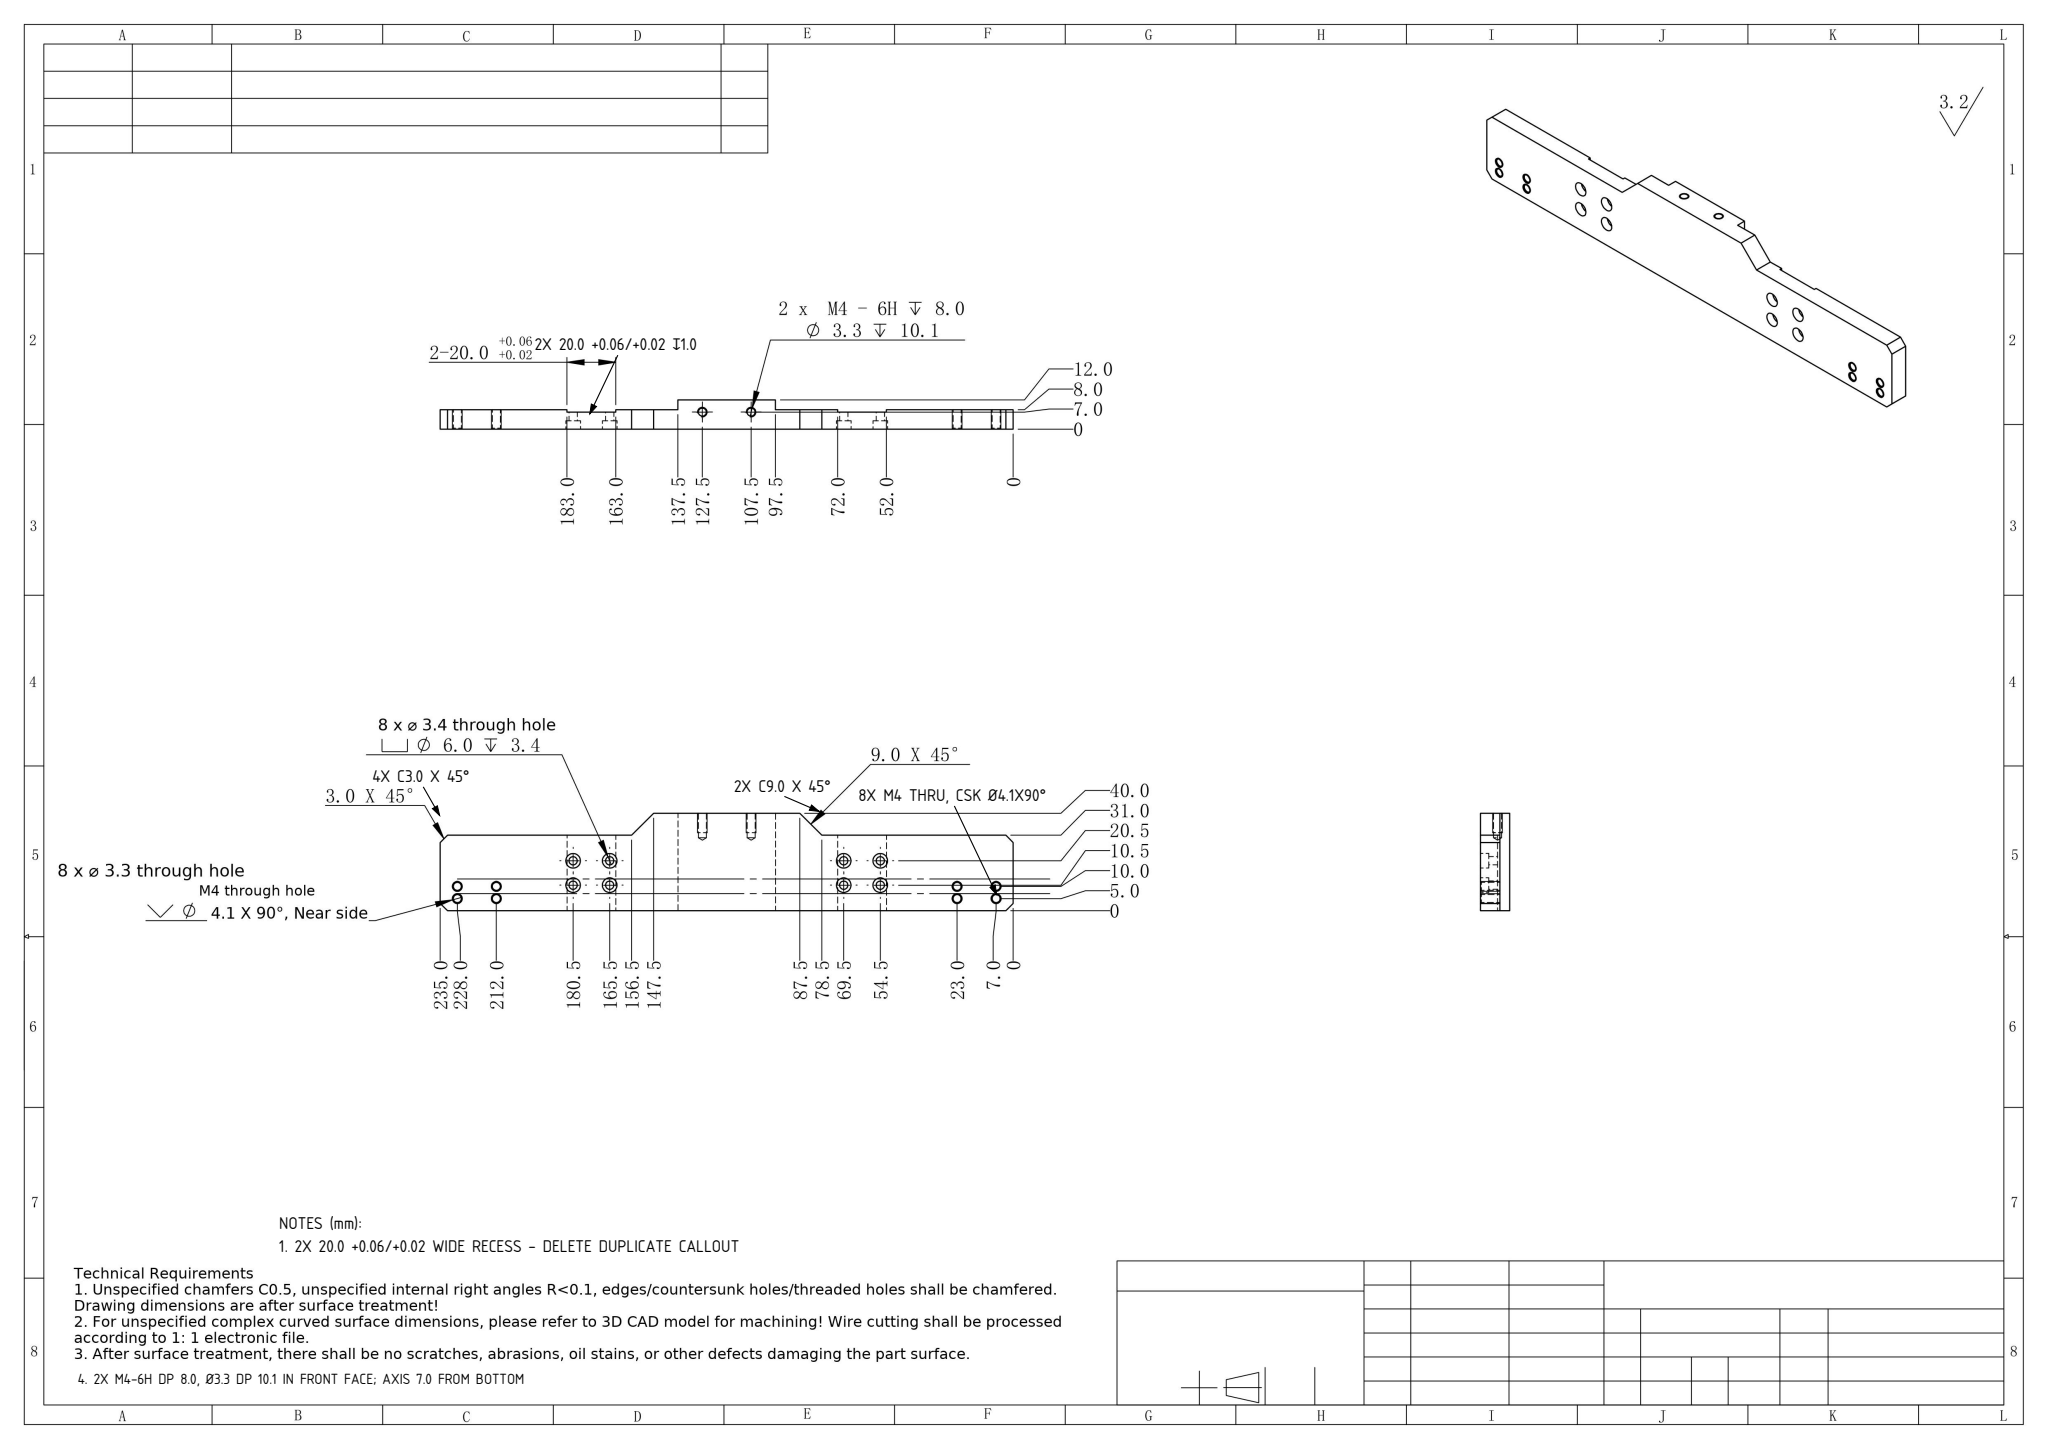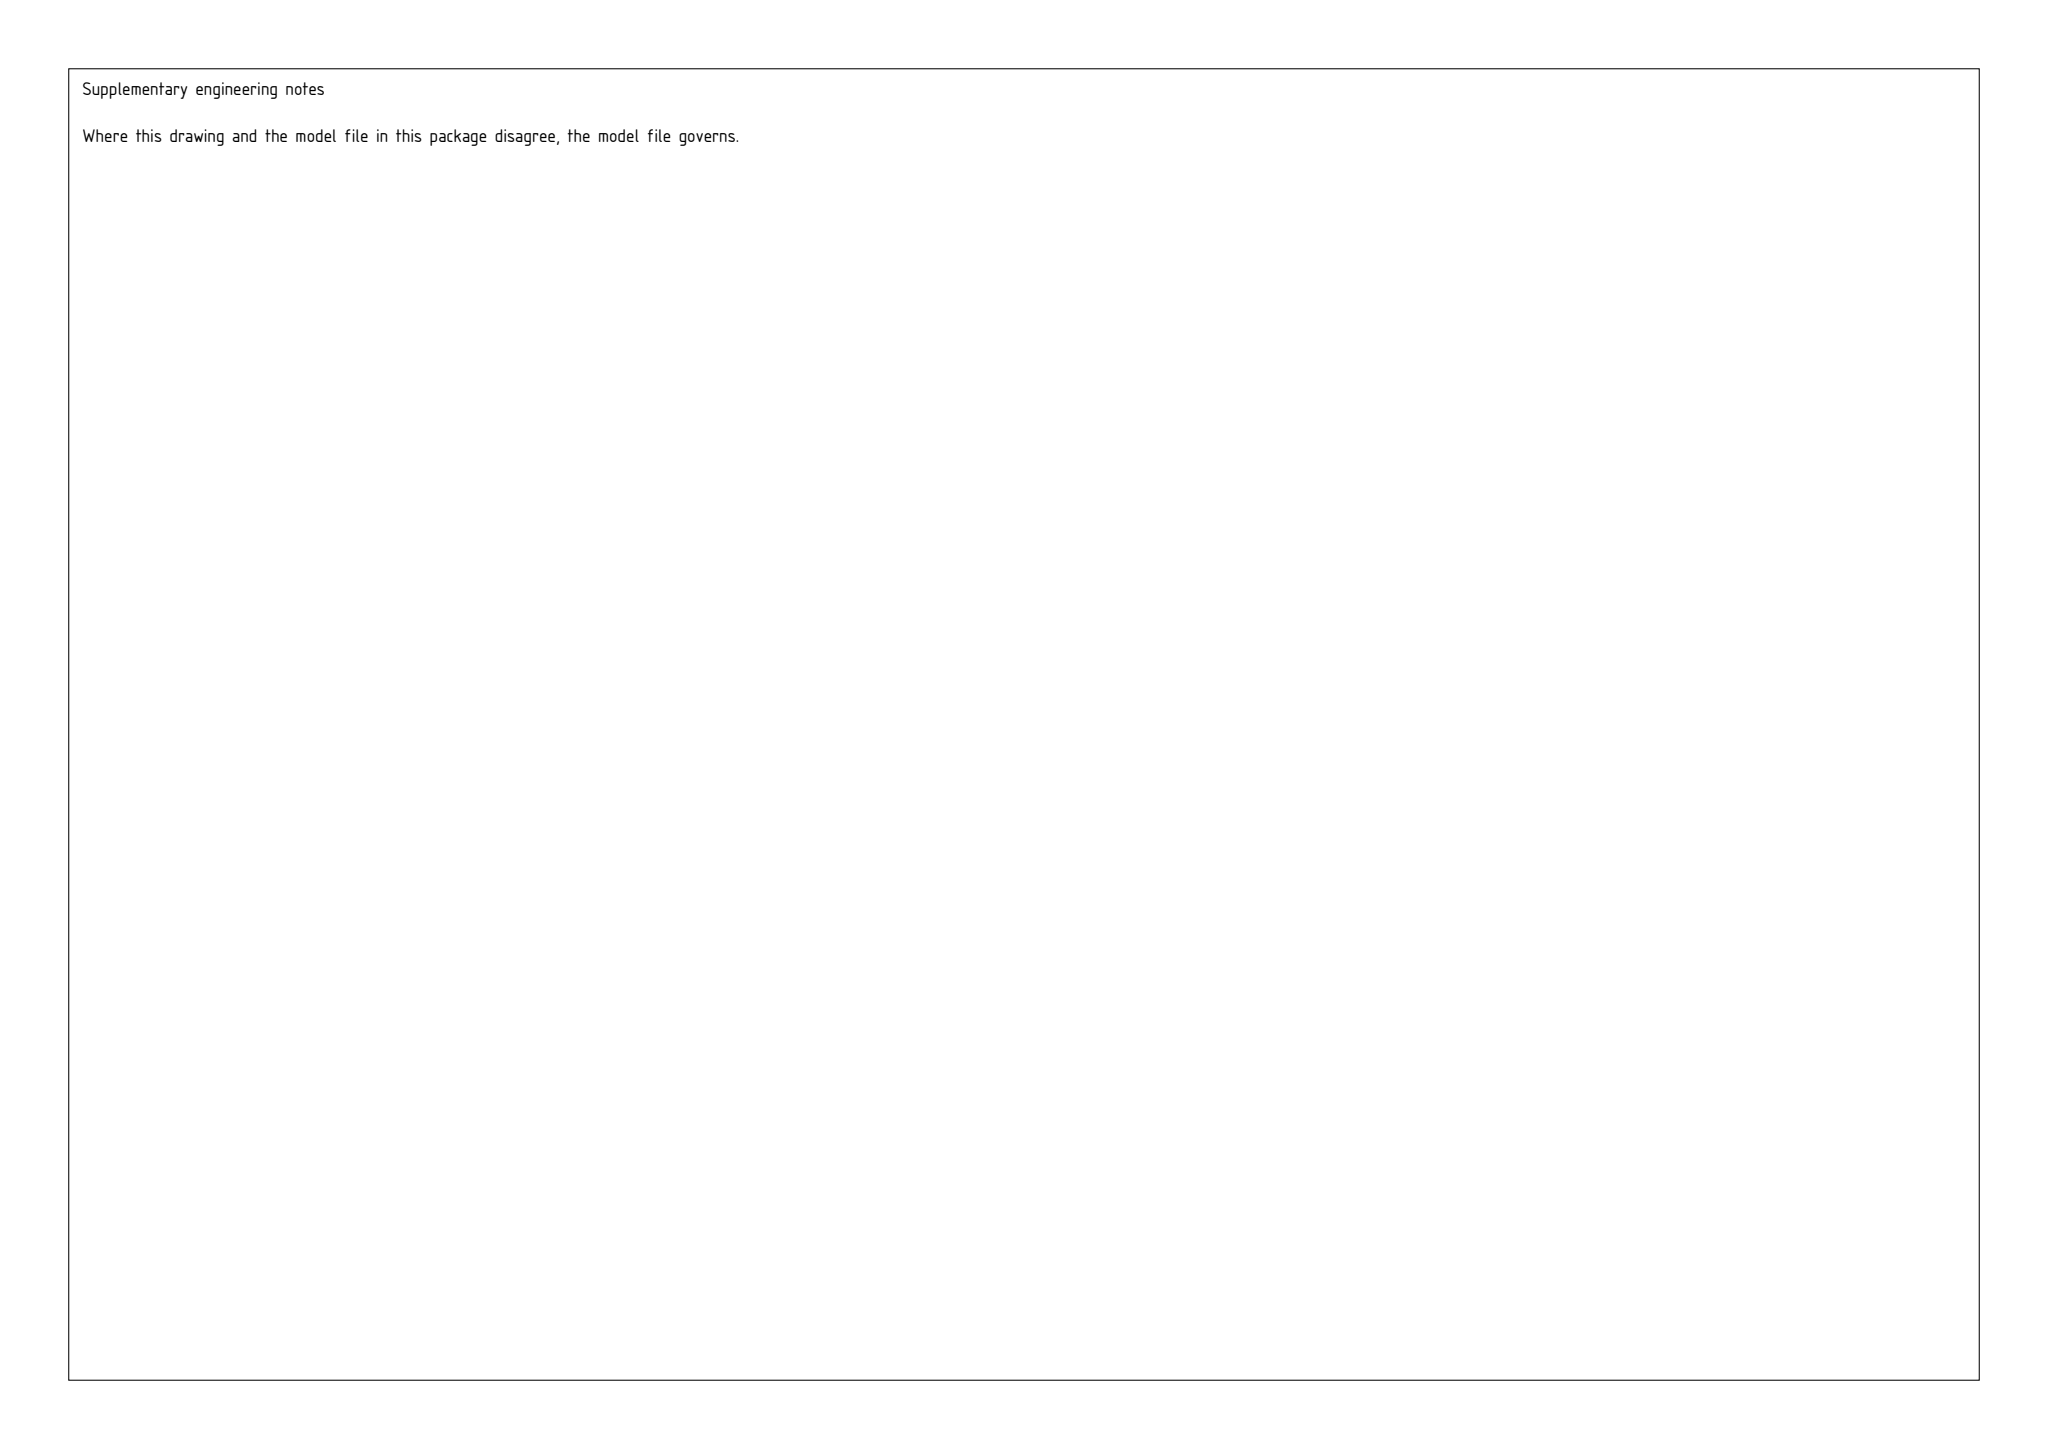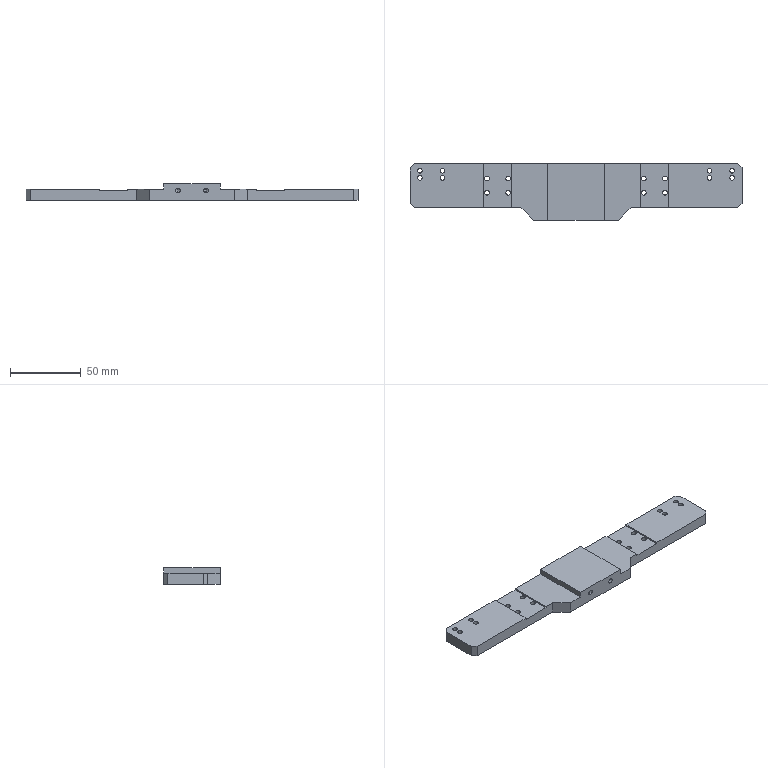Part | SolidWorks | mm | 1 solid | 106 faces | box 235 x 40 x 12 mm | volume 66501 mm3 | cylinder 52 | plane 34 | cone 20 | commonest cylinder face diameters 3.3 x20 6 x16 3.4 x16
Drawing notes:
2X M4-6H DP 8.0, Ø3.3 DP 10.1 IN FRONT FACE; AXIS 7.0 FROM BOTTOM | from the solid: Ø3.3 cyls, axis y, at [107.5,-,7.0] & [127.5,-,7.0], y 0 to 10.1; bottom face z=0
4X 3.0 X 45° CHAMF AT 4 CORNERS, FULL 8.0 HT | from the solid: Inclined 45° faces size 3x3x8 at (0,37),(0,9),(232,37),(232,9)
2X 9.0 X 45° CHAMF ON FRONT FACE, FULL 8.0 HT | from the solid: Inclined 45° faces size 9x9x8 at (147.5,0) and (78.5,0)
2X 20.0 +0.06/+0.02 WIDE RECESS - DELETE DUPLICATE CALLOUT | from the solid: Two recesses 20 wide: x52-72 and x163-183, both z7.0-8.0
2X 20.0 +0.06/+0.02 WIDE X DP 1.0 DEEP, FLOOR Z7.0 FROM BOTTOM | from the solid: z=7.0 faces x[52,72] & x[163,183], y[9,40]; adjacent top face z=8.0
8X M4 THRU (TAP DRILL Ø3.3), CSK Ø4.1 X 90° NEAR SIDE | from the solid: Ø3.3 z-holes at x7,23,212,228 / y30,35 thru to z8.0; 90° cones ref Ø4.05 at z0-0.4